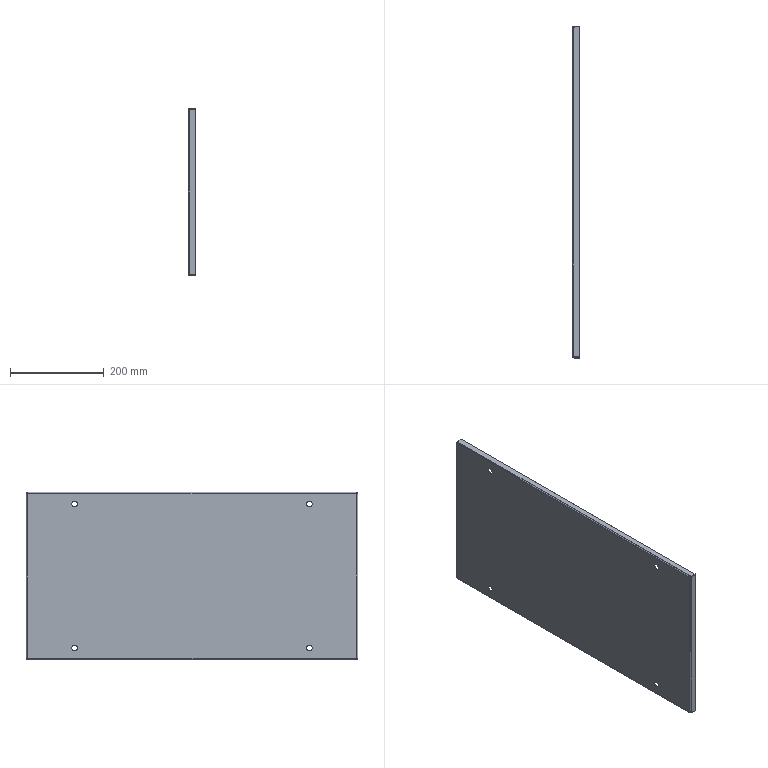Component | SolidWorks | TopCoverPlate-1 | 1 solid | 70 faces | volume 416620 mm3 | plane 54 | cylinder 16 | commonest cylinder face diameters 12 x8 5 x4 2 x4